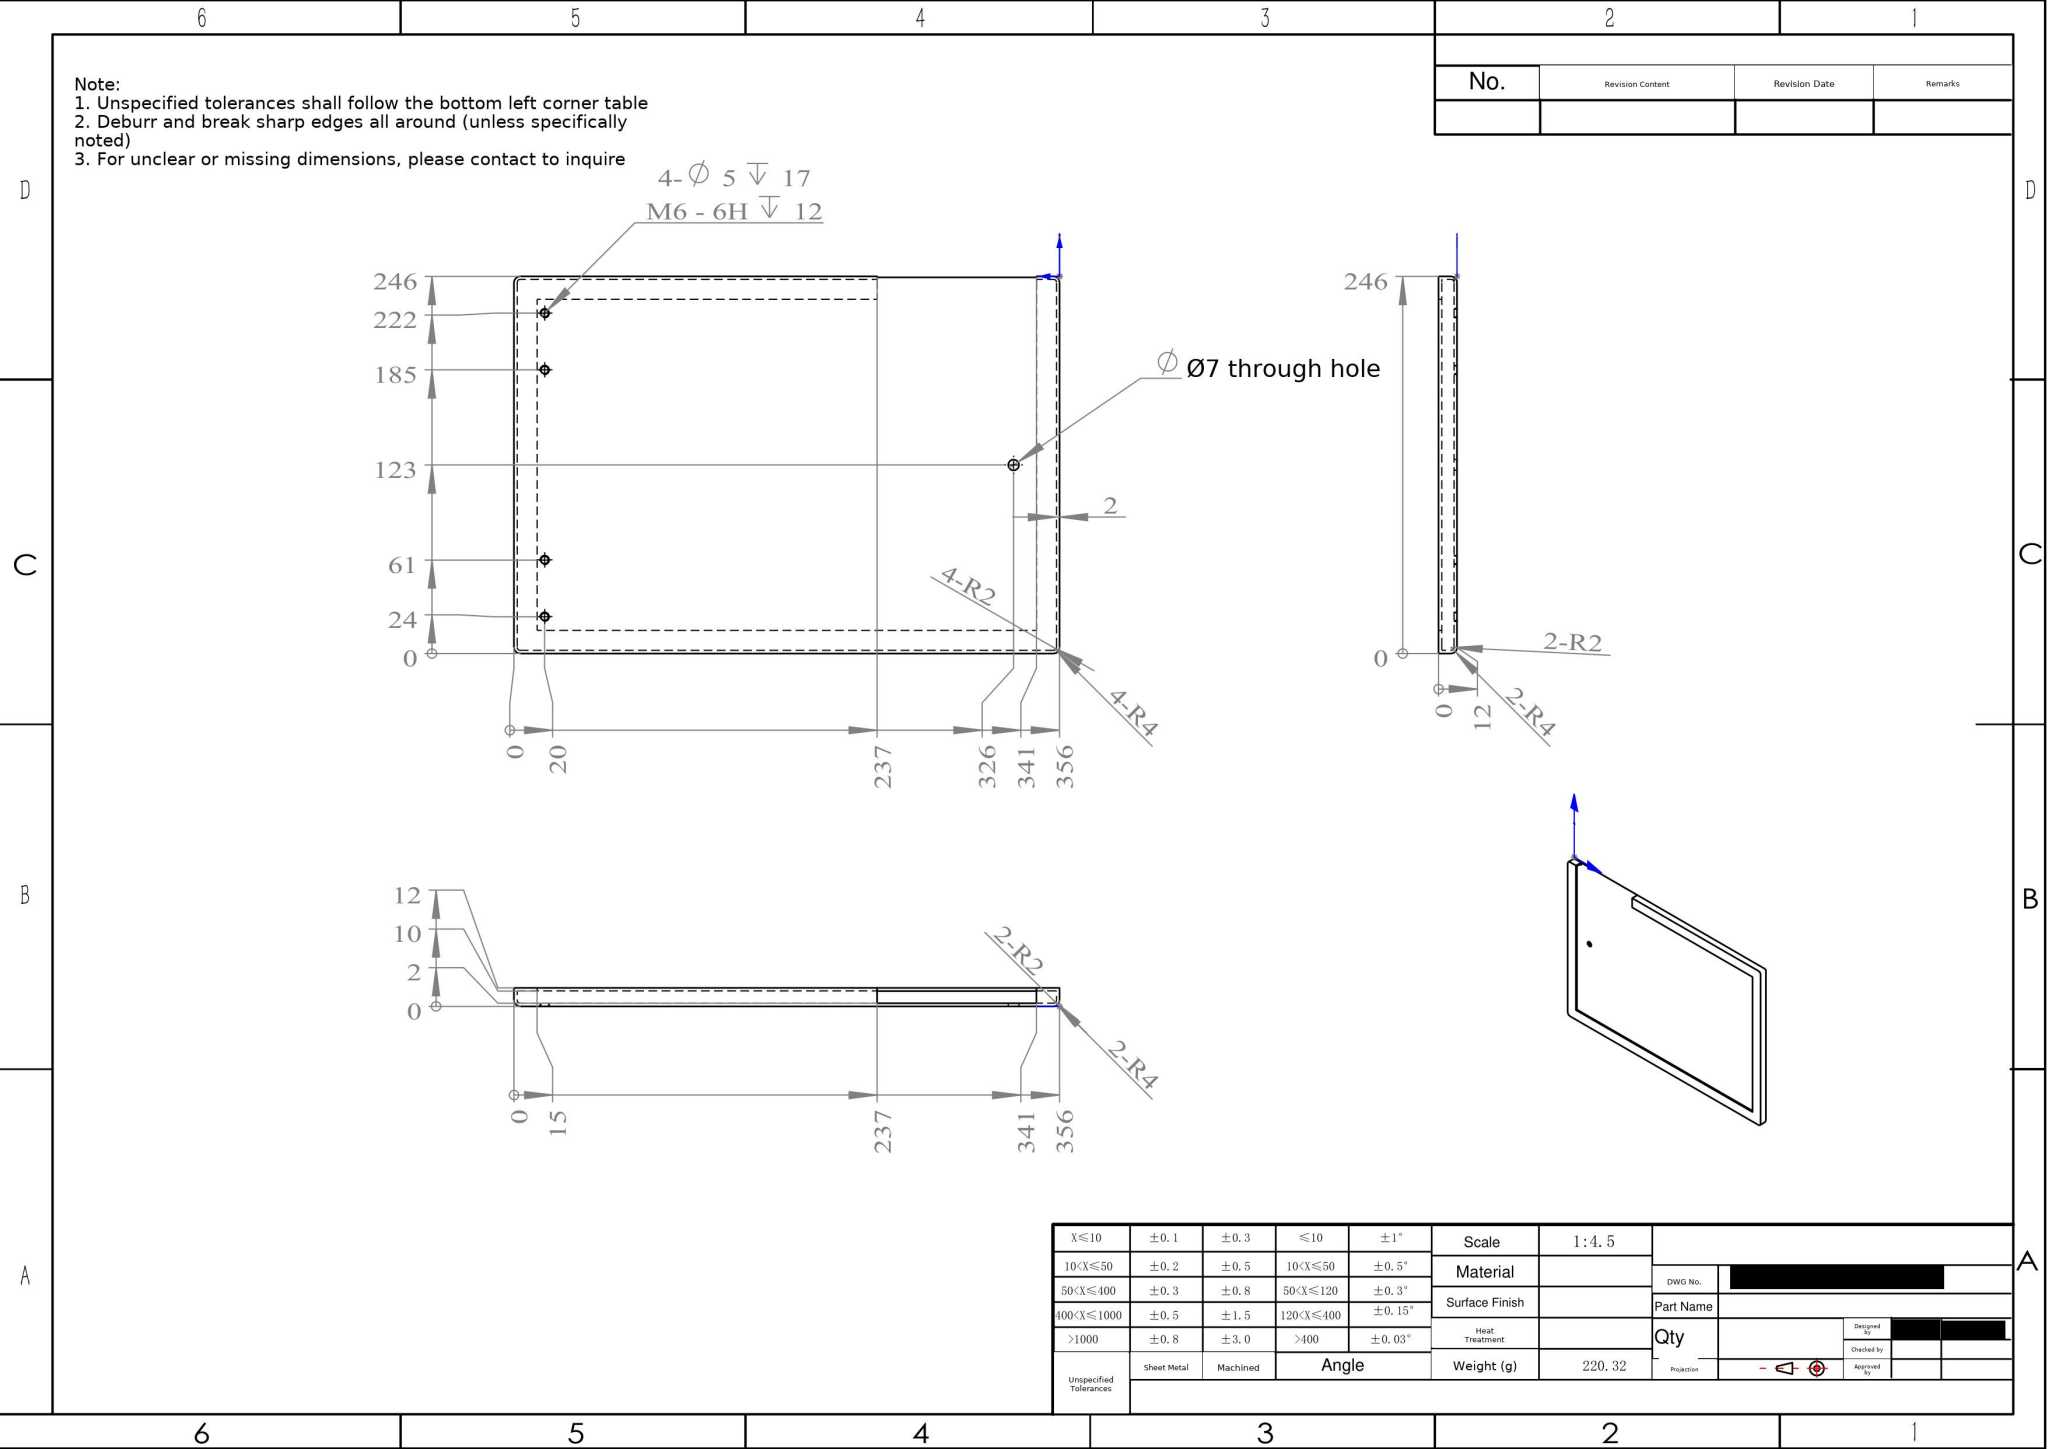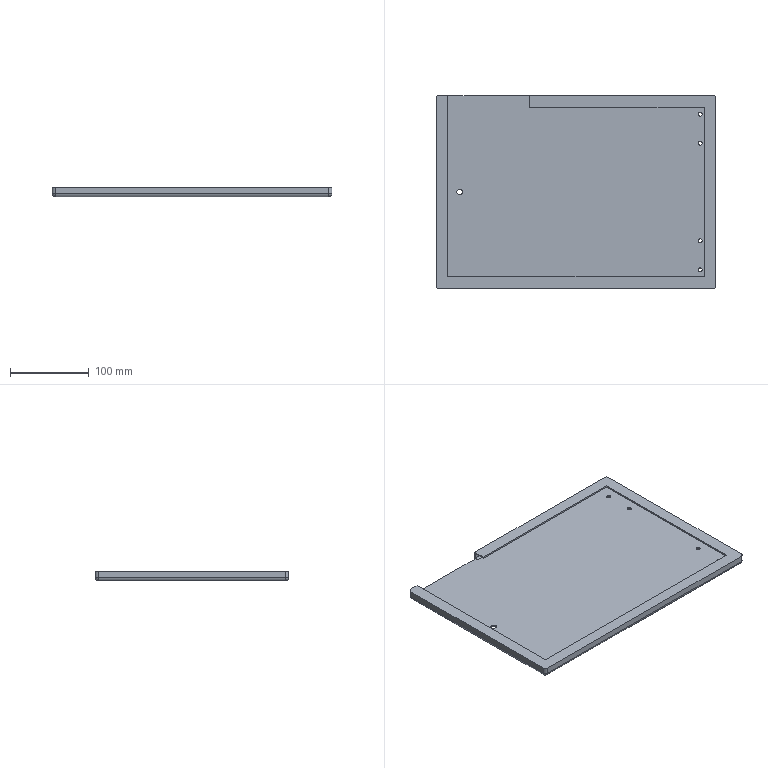Part | SolidWorks | mm | 1 solid | 54 faces | box 356 x 246 x 12 mm | volume 220323 mm3 | cylinder 27 | plane 19 | sphere 8 | commonest cylinder face diameters 4 x9 5 x8 8 x8 7 x2
build123d program:
from build123d import *

# Parameters (mm, degrees)
SKETCH1_W             = 356
SKETCH1_H             = 246
BOSS_EXTRUDE1_DEPTH   = 12
SHELL1_T              = -2
SKETCH3_W             = 356
SKETCH3_H             = 246
SKETCH3_W_2           = 326
SKETCH3_H_2           = 216
BOSS_EXTRUDE2_DEPTH   = 2
FILLET1_R             = 2
FILLET2_R             = 4
SKETCH4_R             = 3.5
CUT_EXTRUDE1_DEPTH    = 433.893
CUT_EXTRUDE2_REACH    = 434.893
SKETCH5_W             = 104
SKETCH5_H             = 15
M6_TAPPED_HOLE1_D     = 5
M6_TAPPED_HOLE1_DEPTH = 17
M6_TAPPED_HOLE1_TIP   = 1.502


with BuildPart() as part:
    # Sketch1 → Boss-Extrude1 (new body)
    with BuildSketch(Plane.XY):
        with Locations((178, -123)):
            Rectangle(SKETCH1_W, SKETCH1_H)
    extrude(amount=BOSS_EXTRUDE1_DEPTH)

    # Shell1
    shell1_openings = [part.faces().sort_by_distance(p)[0] for p in [
        (178, -123, 12),
    ]]
    offset(amount=SHELL1_T, openings=shell1_openings, kind=Kind.INTERSECTION)

    # Sketch3 → Boss-Extrude2 (add)
    with BuildSketch(Plane.XY.offset(12)):
        with Locations((178, -123)):
            Rectangle(SKETCH3_W, SKETCH3_H)
        with Locations((178, -123)):
            Rectangle(SKETCH3_W_2, SKETCH3_H_2, mode=Mode.SUBTRACT)
    extrude(amount=-BOSS_EXTRUDE2_DEPTH)

    # Fillet1
    fillet1_edges = [part.edges().sort_by_distance(p)[0] for p in [
        (354, -123, 2),
        (178, -2, 2),
        (2, -123, 2),
        (178, -244, 2),
        (2, -244, 6),
        (354, -244, 6),
        (2, -2, 6),
        (354, -2, 6),
    ]]
    fillet(fillet1_edges, radius=FILLET1_R)

    # Fillet2
    fillet2_edges = [part.edges().sort_by_distance(p)[0] for p in [
        (178, -246, 0),
        (0, -123, 0),
        (178, 0, 0),
        (356, -123, 0),
        (356, -246, 6),
        (0, -246, 6),
        (0, 0, 6),
        (356, 0, 6),
    ]]
    fillet(fillet2_edges, radius=FILLET2_R)

    # Sketch4 → Cut-Extrude1 (cut, through all)
    with BuildSketch(Plane.XY.offset(12)):
        with Locations((30, -123)):
            Circle(SKETCH4_R)
    extrude(amount=-CUT_EXTRUDE1_DEPTH, mode=Mode.SUBTRACT)

    # Cut-Extrude2: up to this face of the body (flat: up to its plane)
    cut_extrude2_end = Plane(part.part.faces().sort_by_distance((178.069, -123, 2))[0])
    # Sketch5 → Cut-Extrude2 (cut, up to the picked face)
    with BuildSketch(Plane.XY.offset(12), mode=Mode.PRIVATE) as cut_extrude2_sk1:
        with Locations((67, -7.5)):
            Rectangle(SKETCH5_W, SKETCH5_H)
    cut_extrude2_tool1 = split(extrude(cut_extrude2_sk1.sketch, amount=-CUT_EXTRUDE2_REACH, mode=Mode.PRIVATE), bisect_by=cut_extrude2_end, keep=Keep.BOTH, mode=Mode.PRIVATE)
    add(cut_extrude2_tool1.solids().sort_by(Axis((67, -7.5, 12), (0, 0, -1)))[0], mode=Mode.SUBTRACT)

    # M6 Tapped Hole1
    with Locations(Plane(origin=(336, -24, 0), x_dir=(-1, 0, 0), z_dir=(0, 0, -1))):
        with Locations((0, 0), (0, -37), (0, -161), (0, -198)):
            Hole(M6_TAPPED_HOLE1_D / 2, depth=M6_TAPPED_HOLE1_DEPTH)
            with Locations((0, 0, -(M6_TAPPED_HOLE1_DEPTH + M6_TAPPED_HOLE1_TIP / 2))):  # 118° drill point
                Cone(0, M6_TAPPED_HOLE1_D / 2, M6_TAPPED_HOLE1_TIP, mode=Mode.SUBTRACT)


solid = part.part